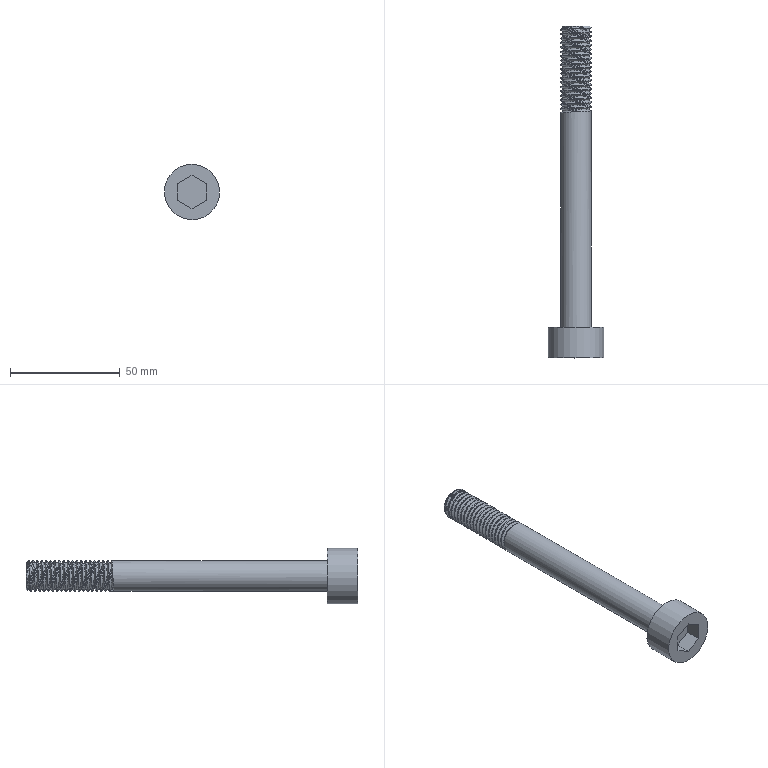Component | NX | ALLINE_SCREW_M14_BP_2_DP_2 | 1 solid | 37 faces | volume 26087 mm3 | cylinder 22 | plane 12 | spline 2 | cone 1 | commonest cylinder face diameters 14 x20 25.2 x1 12 x1